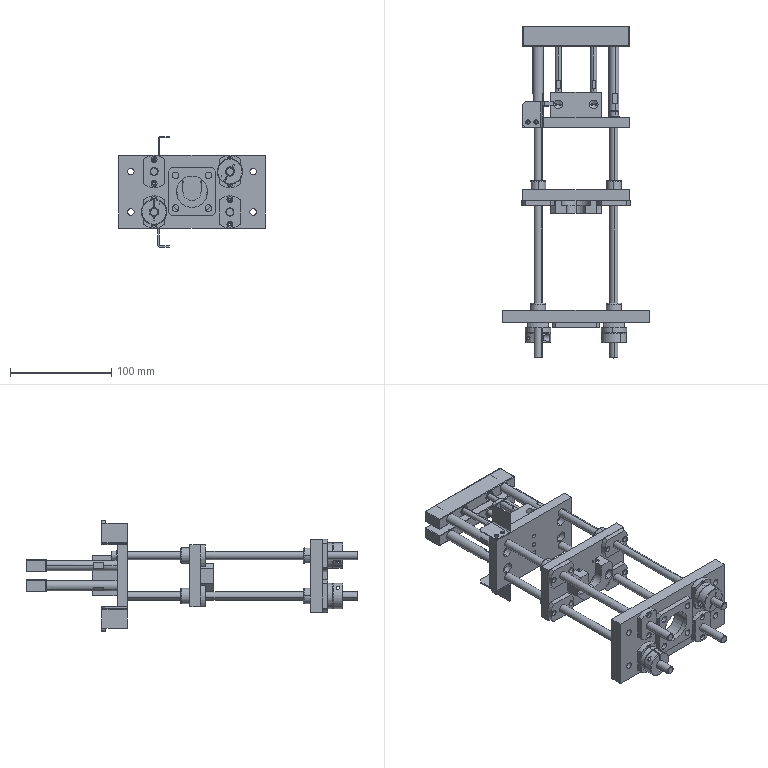Assembly | SolidWorks | mm | 38 component files | 38 solids | 1015 faces | box 145 x 328 x 109.5 mm | volume 440612 mm3 | cylinder 514 | plane 343 | cone 126 | sphere 16 | spline 16 | commonest cylinder face diameters 5 x54 10 x44 6 x42 2.5 x40 8 x38 6.6 x32 11 x32 15 x32
Bill of materials:
F12529-M1072 | 2 |  | Thick annular ring with a central through bore, a single radial slit cutting through one side of the ring, and chamfered outer edges; resembles a one-piece split collar.
F12529-M1073 | 2 |  | Plain flat annular disc (washer- or spacer-like) with a single concentric through hole and square edges.
F12529-M5101 | 1 |  | Rectangular flat plate with a symmetric through-hole pattern: one large central hole, four medium holes in a rectangular pattern, four smaller holes around the central hole, four holes near the short edges, and eight small holes paired above and below the medium holes.
F12529-M5102 | 1 |  | Rectangular flat plate with two columns of four through holes near each short end, three smaller holes in a central vertical line, and two holes drilled into one narrow edge face.
F12529-M5103 | 1 |  | Rectangular flat plate with four large through holes near the corners, each flanked by two small holes, plus a central group of two medium holes and four small holes in a rectangular pattern.
F12529-M5104 | 2 |  | Long rectangular bar with four holes through one long side face: two larger plain holes inboard and two smaller holes outboard that appear counterbored; edges carry small rounds or chamfers.
F12529-M5105 | 4 |  | Slender cylindrical tube/rod with an axial bore and a short flat machined on one side partway along its length.
F12529-M5106 | 4 | AISI 304 | Stepped cylindrical shaft with reduced-diameter journals at both ends, a slightly larger main body with a subtle step, a small groove near one end, and a small axial through bore.
F12529-M5107 | 1 | AISI 304 | Solid rectangular block with two through holes from the top face and two smaller holes on one side face that appear blind with conical bottoms.
F12529-M5112 | 1 |  | Block with chamfered (octagon-like) corners and a central U-shaped slot with a semicircular bottom open to one edge, with two round through holes on either side of the slot; the tops of the uprights have a stepped rebate.
F12529-M5116 | 1 |  | Square flat flange-style plate with chamfered corners, a large central through hole, and four smaller through holes near the corners.
F12529-S5108 | 1 |  | Sheet-metal Z-shaped bracket: a base flange with two round holes and chamfered corners, a vertical web, and a narrower top tab bent in the opposite direction.
F12529-S5109 | 1 |  | Bent sheet-like bracket in a Z/offset profile: an upper flange with two round through-holes, a vertical web joined by a radiused bend, and a narrower lower tab bent the opposite way from the web.
LBH8 | 8 |  | Flanged cylindrical bushing/boss: a flat flange shaped like a circle with two straight-cut sides, two small through-holes in the flange, and a central bore through a cylindrical boss.
SCB5-20 | 2 |  | Headed cylindrical pin or fastener-like body: a short cylindrical head with a larger diameter on a long plain cylindrical shank.
SSPWF5 | 2 |  | Plain flat annular ring (washer-like): a thin disc with a concentric central through-hole.
SFJT8-230-M5 | 4 |  | Long slender solid cylindrical rod with flat ends.
Mates:
1. distance | F12529-M5102-1 face at (-52.5, 203, 30.5) dir (0, 1, 0) | F12529-M5104-1 face at (-52.5, 273, 16) dir (0, -1, 0)
2. distance | F12529-M5102-1 face at (-52.5, 203, 30.5) dir (0, 1, 0) | F12529-M5104-2 face at (-52.5, 273, -4) dir (0, -1, 0)
3. coincident | F12529-M5104-1 face at (52.5, 273, 16) dir (1, 0, 0) | F12529-M5104-2 face at (52.5, 273, -4) dir (1, 0, 0)
4. parallel | F12529-M5102-1 face at (-52.5, 203, 30.5) dir (0, 0, 1) | F12529-M5104-1 face at (-52.5, 293, 16) dir (0, 0, 1)
5. parallel | F12529-M5102-1 face at (-52.5, 203, -30.5) dir (0, 0, -1) | F12529-M5104-2 face at (-52.5, 293, -16) dir (0, 0, -1)
6. coincident | F12529-M5102-1 face at (-52.5, 203, -30.5) dir (-1, 0, 0) | F12529-M5104-1 face at (-52.5, 273, 16) dir (-1, 0, 0)
7. concentric | F12529-M5101-1 face at (-37.5, 0, 20) dir (0, 1, 0) r 7.5 | LBH8-9 face at (-37.5, 9.625, 20) dir (0, 1, 0) r 7.5
8. coincident | F12529-M5101-1 face at (-72.5, 0, 36) dir (0, -1, 0) | LBH8-9 face at (-37.5, 0, 8.4) dir (0, 1, 0)
9. concentric | F12529-M5101-1 face at (-37.5, 0, -20) dir (0, 1, 0) r 7.5 | LBH8-12 face at (-37.5, 9.625, -20) dir (0, 1, 0) r 7.5
10. coincident | F12529-M5101-1 face at (-72.5, 0, 36) dir (0, -1, 0) | LBH8-12 face at (-37.5, 0, -8.4) dir (0, 1, 0)
11. concentric | F12529-M5101-1 face at (37.5, 0, 20) dir (0, 1, 0) r 7.5 | LBH8-11 face at (37.5, 9.625, 20) dir (0, 1, 0) r 7.5
12. coincident | F12529-M5101-1 face at (-72.5, 0, 36) dir (0, -1, 0) | LBH8-11 face at (37.5, 0, 31.6) dir (0, 1, 0)
13. concentric | F12529-M5101-1 face at (37.5, 0, -20) dir (0, 1, 0) r 7.5 | LBH8-10 face at (37.5, 9.625, -20) dir (0, 1, 0) r 7.5
14. coincident | F12529-M5101-1 face at (-72.5, 0, 36) dir (0, -1, 0) | LBH8-10 face at (37.5, 0, -8.4) dir (0, 1, 0)
15. distance | F12529-M5102-1 face at (-52.5, 203, 30.5) dir (0, 0, 1) | F12529-M5104-1 face at (-52.5, 293, 16) dir (0, 0, 1)
16. distance | F12529-M5102-1 face at (-52.5, 203, -30.5) dir (0, 0, -1) | F12529-M5104-2 face at (-52.5, 293, -16) dir (0, 0, -1)
17. parallel | F12529-M5101-1 face at (-72.5, 12, 36) dir (0, 0, 1) | F12529-M5103-1 face at (-52.5, 131, 30.5) dir (0, 0, 1)
18. concentric | F12529-M5102-1 face at (-37.5, 201, 10) dir (0, 1, 0) r 5 | F12529-M5105-1 face at (-37.5, 275, 10) dir (0, -1, 0) r 5
19. coincident | F12529-M5102-1 face at (-37.5, 201, 10) dir (0, 1, 0) | F12529-M5105-1 face at (-37.5, 201, 10) dir (0, -1, 0)
20. coincident | F12529-M5102-1 face at (-37.5, 201, -10) dir (0, 1, 0) | F12529-M5105-2 face at (-37.5, 201, -10) dir (0, -1, 0)
21. concentric | F12529-M5102-1 face at (-37.5, 201, -10) dir (0, 1, 0) r 5 | F12529-M5105-2 face at (-37.5, 275, -10) dir (0, -1, 0) r 5
22. concentric | F12529-M5102-1 face at (37.5, 201, -10) dir (0, 1, 0) r 5 | F12529-M5105-3 face at (37.5, 275, -10) dir (0, -1, 0) r 5
23. coincident | F12529-M5102-1 face at (37.5, 201, -10) dir (0, 1, 0) | F12529-M5105-3 face at (37.5, 201, -10) dir (0, -1, 0)
24. coincident | F12529-M5102-1 face at (37.5, 201, 10) dir (0, 1, 0) | F12529-M5105-4 face at (37.5, 201, 10) dir (0, -1, 0)
25. concentric | F12529-M5102-1 face at (37.5, 201, 10) dir (0, 1, 0) r 5 | F12529-M5105-4 face at (37.5, 275, 10) dir (0, -1, 0) r 5
26. parallel | F12529-M5101-1 face at (-72.5, 12, -36) dir (-1, 0, 0) | LBH8-9 face at (-48, -5, 7.927) dir (-1, 0, 0)
27. parallel | F12529-M5101-1 face at (-72.5, 12, -36) dir (-1, 0, 0) | LBH8-12 face at (-48, -5, -32.073) dir (-1, 0, 0)
28. parallel | F12529-M5101-1 face at (72.5, 12, -36) dir (1, 0, 0) | LBH8-11 face at (48, -5, 32.073) dir (1, 0, 0)
29. parallel | F12529-M5101-1 face at (72.5, 12, -36) dir (1, 0, 0) | LBH8-10 face at (48, -5, -7.927) dir (1, 0, 0)
30. concentric | F12529-M5106-1 face at (-17.5, 219.5, 10) dir (0, 1, 0) r 2.5 | F12529-M5107-1 face at (-17.5, 227.5, 10) dir (0, 1, 0) r 2.5
31. coincident | F12529-M5106-1 face at (-17.5, 227.5, 10) dir (0, -1, 0) | F12529-M5107-1 face at (-25, 227.5, 20) dir (0, 1, 0)
32. parallel | F12529-M5102-1 face at (-52.5, 203, 30.5) dir (0, 0, 1) | F12529-M5107-1 face at (-25, 227.5, 20) dir (0, 0, 1)
33. concentric | F12529-M5103-1 face at (37.5, 121, -20) dir (0, 1, 0) r 7.5 | LBH8-13 face at (37.5, 130.625, -20) dir (0, 1, 0) r 7.5
34. coincident | F12529-M5103-1 face at (-52.5, 121, -30.5) dir (0, -1, 0) | LBH8-13 face at (49.1, 121, -20) dir (0, 1, 0)
35. coincident | F12529-M5103-1 face at (-52.5, 131, -30.5) dir (0, 0, -1) | LBH8-13 face at (49.573, 116, -30.5) dir (0, 0, -1)
36. concentric | F12529-M5103-1 face at (37.5, 121, 20) dir (0, 1, 0) r 7.5 | LBH8-14 face at (37.5, 130.625, 20) dir (0, 1, 0) r 7.5
37. coincident | F12529-M5103-1 face at (-52.5, 121, -30.5) dir (0, -1, 0) | LBH8-14 face at (49.1, 121, 20) dir (0, 1, 0)
38. coincident | F12529-M5103-1 face at (-52.5, 121, -30.5) dir (0, -1, 0) | LBH8-15 face at (-25.9, 121, 20) dir (0, 1, 0)
39. coincident | F12529-M5103-1 face at (-52.5, 131, 30.5) dir (0, 0, 1) | LBH8-15 face at (-49.573, 116, 30.5) dir (0, 0, 1)
40. coincident | F12529-M5103-1 face at (-52.5, 121, -30.5) dir (0, -1, 0) | LBH8-16 face at (-25.9, 121, -20) dir (0, 1, 0)
41. coincident | F12529-M5103-1 face at (-52.5, 131, -30.5) dir (0, 0, -1) | LBH8-16 face at (-25.427, 116, -30.5) dir (0, 0, -1)
42. coincident | F12529-M5103-1 face at (-52.5, 131, 30.5) dir (0, 0, 1) | LBH8-14 face at (25.427, 116, 30.5) dir (0, 0, 1)
43. coincident | F12529-M5102-1 face at (-52.5, 203, 30.5) dir (0, 0, 1) | F12529-S5108-2 face at (-52.5, 218, 30.5) dir (0, 0, -1)
44. coincident | F12529-M5102-1 face at (-52.5, 203, -30.5) dir (-1, 0, 0) | F12529-S5108-2 face at (-52.5, 218, 31.5) dir (-1, 0, 0)
45. coincident | F12529-M5102-1 face at (-52.5, 203, -30.5) dir (0, 0, -1) | F12529-S5109-1 face at (-52.5, 193, -30.5) dir (0, 0, 1)
46. coincident | F12529-M5102-1 face at (-52.5, 203, -30.5) dir (-1, 0, 0) | F12529-S5109-1 face at (-52.5, 193, -32) dir (-1, 0, 0)
47. concentric | SFJT8-230-M5-4 face at (37.5, -35, 20) dir (0, 1, 0) r 4 | F12529-M5102-1 face at (37.5, 195, 20) dir (0, -1, 0) r 4
48. coincident | SFJT8-230-M5-4 face at (37.5, 195, 20) dir (0, 1, 0) | F12529-M5102-1 face at (37.5, 195, 20) dir (0, -1, 0)
49. concentric | SFJT8-230-M5-4 face at (37.5, -35, 20) dir (0, 1, 0) r 4 | LBH8-14 face at (37.5, 128, 20) dir (0, 1, 0) r 4
50. concentric | SFJT8-230-M5-3 face at (37.5, -35, -20) dir (0, 1, 0) r 4 | F12529-M5102-1 face at (37.5, 195, -20) dir (0, -1, 0) r 4
51. concentric | SFJT8-230-M5-4 face at (37.5, -35, 20) dir (0, 1, 0) r 4 | LBH8-11 face at (37.5, 7, 20) dir (0, 1, 0) r 4
52. concentric | SFJT8-230-M5-1 face at (-37.5, -35, 20) dir (0, 1, 0) r 4 | F12529-M5102-1 face at (-37.5, 195, 20) dir (0, -1, 0) r 4
53. coincident | SFJT8-230-M5-1 face at (-37.5, 195, 20) dir (0, 1, 0) | F12529-M5102-1 face at (-37.5, 195, 20) dir (0, -1, 0)
54. concentric | SFJT8-230-M5-1 face at (-37.5, -35, 20) dir (0, 1, 0) r 4 | LBH8-15 face at (-37.5, 128, 20) dir (0, 1, 0) r 4
55. coincident | SFJT8-230-M5-3 face at (37.5, 195, -20) dir (0, 1, 0) | F12529-M5102-1 face at (37.5, 195, -20) dir (0, -1, 0)
56. coincident | SFJT8-230-M5-2 face at (-37.5, 195, -20) dir (0, 1, 0) | F12529-M5102-1 face at (-37.5, 195, -20) dir (0, -1, 0)
57. concentric | SFJT8-230-M5-2 face at (-37.5, -35, -20) dir (0, 1, 0) r 4 | F12529-M5102-1 face at (-37.5, 195, -20) dir (0, -1, 0) r 4
58. concentric | SFJT8-230-M5-2 face at (-37.5, -35, -20) dir (0, 1, 0) r 4 | LBH8-16 face at (-37.5, 128, -20) dir (0, 1, 0) r 4
59. coincident | F12529-M5102-1 face at (-52.5, 203, 30.5) dir (0, 1, 0) | M5Screw-1/SSPWF5-1 face at (39.806, 203, 19.034) dir (0, -1, 0)
60. concentric | F12529-M5102-1 face at (37.5, 193, 20) dir (0, 1, 0) r 2.75 | M5Screw-1/SCB5-20-1 face at (37.5, 194.245, 20) dir (0, -1, 0) r 2.5
61. coincident | F12529-M5102-1 face at (-52.5, 203, 30.5) dir (0, 1, 0) | M5Screw-2/SSPWF5-1 face at (-35, 203, 20) dir (0, -1, 0)
62. concentric | F12529-M5102-1 face at (-37.5, 193, 20) dir (0, 1, 0) r 2.75 | M5Screw-2/SCB5-20-1 face at (-37.5, 194.245, 20) dir (0, -1, 0) r 2.5
63. coincident | F12529-M5103-1 face at (-52.5, 121, -30.5) dir (0, -1, 0) | F12529-M5112-1 face at (25, 121, -18) dir (0, 1, 0)
64. parallel | F12529-M5103-1 face at (-52.5, 131, 30.5) dir (0, 0, 1) | F12529-M5112-1 face at (25, 121, 12) dir (0, 0, 1)
65. concentric | SFJT8-230-M5-4 face at (37.5, -35, 20) dir (0, 1, 0) r 4 | F12529-M1072-1 face at (37.5, -10, 20) dir (0, -1, 0) r 4
66. concentric | SFJT8-230-M5-4 face at (37.5, -35, 20) dir (0, 1, 0) r 4 | F12529-M1073-1 face at (37.5, -5, 20) dir (0, -1, 0) r 4.5
67. coincident | LBH8-11 face at (37.5, -5, 30) dir (0, -1, 0) | F12529-M1073-1 face at (37.5, -5, 20) dir (0, 1, 0)
68. coincident | F12529-M1072-1 face at (37.5, -10, 20) dir (0, 1, 0) | F12529-M1073-1 face at (37.5, -10, 20) dir (0, -1, 0)
69. concentric | SFJT8-230-M5-2 face at (-37.5, -35, -20) dir (0, 1, 0) r 4 | F12529-M1073-2 face at (-37.5, -5, -20) dir (0, -1, 0) r 4.5
70. coincident | LBH8-12 face at (-37.5, -5, -10) dir (0, -1, 0) | F12529-M1073-2 face at (-37.5, -5, -20) dir (0, 1, 0)
71. coincident | F12529-M1073-2 face at (-37.5, -10, -20) dir (0, -1, 0) | F12529-M1072-2 face at (-37.5, -10, -20) dir (0, 1, 0)
72. concentric | SFJT8-230-M5-2 face at (-37.5, -35, -20) dir (0, 1, 0) r 4 | F12529-M1072-2 face at (-37.5, -10, -20) dir (0, -1, 0) r 4
73. coincident | F12529-M5102-1 face at (-52.5, 193, 30.5) dir (0, -1, 0) | F12529-S5109-1 face at (-31, 193, -52) dir (0, -1, 0)
74. coincident | F12529-M5102-1 face at (-52.5, 193, 30.5) dir (0, -1, 0) | F12529-S5108-2 face at (-33.5, 193, 33) dir (0, -1, 0)
75. concentric | SCB5-20-1 face at (9.755, 0, 0) dir (1, 0, 0) r 2.5 | SSPWF5-1 face at (0.5, 0, 0) dir (1, 0, 0) r 2.65
76. coincident | SCB5-20-1 face at (0, 3.375, 0) dir (1, 0, 0) | SSPWF5-1 face at (0, 2.5, 0) dir (-1, 0, 0)